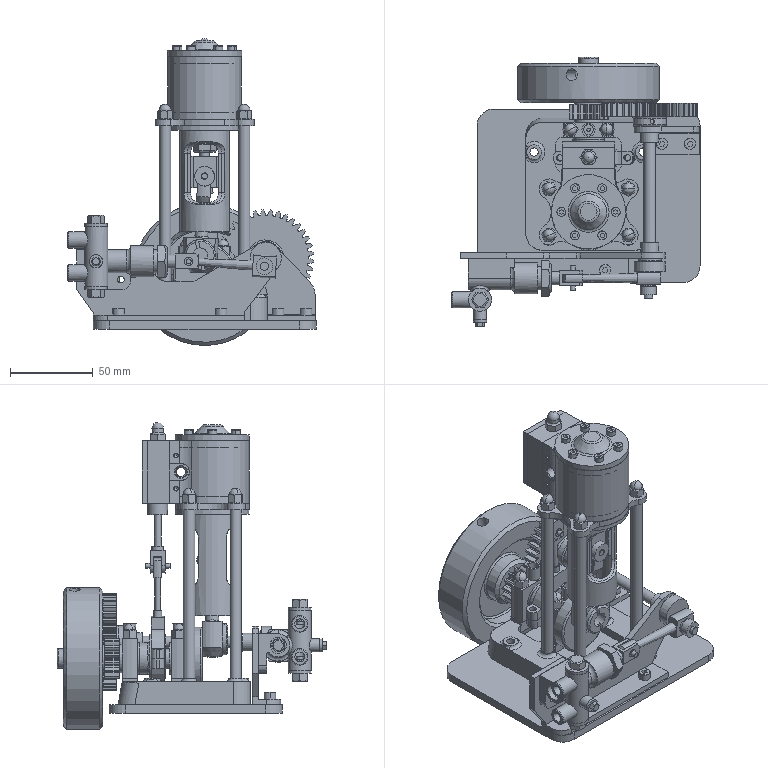Assembly | NX | mm | 88 component files | 88 solids | 1687 faces | box 150.23 x 163.5 x 186 mm | volume 461550 mm3 | plane 696 | cylinder 542 | other 255 | cone 98 | torus 67 | sphere 19 | spline 10 | commonest cylinder face diameters 4 x54 5 x50 51.75 x37 6 x30 14 x27 3 x24 2.5 x22 7 x21
Bill of materials:
unnamed part 1 | 1 |  | Short cylindrical disc/wheel with chamfered outer edges, an annular recess in one face, a raised central hub with a through-bore, and a small radial hole in the outer rim.
unnamed part 2 | 1 |  | Flanged cylindrical sleeve: a short tube with a larger-diameter flange at one end and a straight through-bore.
unnamed part 3 | 2 |  | Stepped hollow cylinder: a larger-diameter tube section with a rounded shoulder that steps down to a smaller-diameter section. It has a large bore at the large end and a smaller hole visible at the opposite end.
unnamed part 4 | 1 |  | Thin sheet-metal-like band formed into an open circular loop, with two parallel straight flanges extending from the opening. Each flange has an open-ended U-shaped slot between two small round holes.
unnamed part 5 | 1 |  | Semicircular saddle/arch body with a flat lug at each end and a rectangular block on top of the arch. Each end lug has a through-hole with rounded ends, and the top block has a vertical hole.
unnamed part 6 | 1 |  | Solid stepped round pin/shaft: a long central body with a smaller-diameter journal of similar length at each end, and small chamfers or rounds at the shoulders.
unnamed part 7 | 1 |  | Link/rod with a rectangular eye block at each end joined by a slightly tapered round shank. The two end blocks have through-holes of different sizes, and the larger block has a short raised ring/boss around its hole on the sides.
unnamed part 8 | 1 |  | Flat annular ring/washer with a uniform rectangular cross-section and a central through-hole.
unnamed part 9 | 1 |  | Long thin-walled tube with a short reduced-diameter spigot step at one end.
unnamed part 10 | 2 |  | Rectangular block with a large through-bore through its main face and three holes in the top face (two smaller outer holes and a larger center hole). Its short end faces are slightly curved.
unnamed part 11 | 4 |  | Cap-screw-shaped part: a cylindrical head with a hexagonal socket recess and a smaller plain cylindrical shank with a chamfered tip.
unnamed part 12 | 1 |  | Rod-end/link with a forked clevis at one end (two lugs, each with a small cross-hole) joined by a tapered shank to a block at the other end. The block has a large through-bore and a chamfered/rounded bottom.
unnamed part 13 | 1 |  | Solid stepped cylindrical shaft: a larger central cylinder with a smaller coaxial cylindrical journal at each end, roughly symmetric.
unnamed part 14 | 1 |  | Thin-walled cylindrical tube with a flat circular flange at one end. The flange has four evenly spaced small holes, and two opposite rounded-rectangle windows are cut through the tube wall.
unnamed part 15 | 1 |  | Flanged bushing: a cylindrical shank joined to a hexagonal collar, with a coaxial through bore. The outer face of the hex is chamfered or crowned.
unnamed part 16 | 1 |  | Long, slender stepped pin: a longer central cylindrical section of slightly larger diameter, with a shorter, narrower cylindrical section at each end. The ends appear rounded or chamfered.
unnamed part 17 | 4 |  | Plain solid cylindrical rod with flat ends.
unnamed part 18 | 1 |  | Circular flange plate with six evenly spaced through holes and a raised central conical boss with a flat, rounded-edge top. The underside has a shallow circular spigot or step.
unnamed part 19 | 1 |  | Flat plate with a lobed outline: four rounded corner ears, each with a larger hole, plus four smaller holes further inboard. There is a central through hole, a thin raised circular pad on the top face, and a cylindrical hub projecting from the underside.
unnamed part 20 | 1 |  | Hex-based tubular fitting: a hexagonal base with a taller cylindrical tubular boss and a coaxial through bore. The bottom edges of the hex are rounded or chamfered.
unnamed part 21 | 1 |  | Half-round saddle clamp: a semicircular band with a flat tab at each end, each tab having a through hole.
unnamed part 22 | 1 |  | Plain cylindrical tube or ring spacer with a concentric through bore and flat ends.
unnamed part 23 | 1 |  | Clevis-style block: a rectangular body with a U-shaped slot forming two prongs. The prongs have rounded ends and one coaxial cross hole through both. A cylindrical boss with an axial hole sits on the opposite face.
unnamed part 24 | 1 |  | Cylindrical housing with a large through bore and a flange at each end. Six small holes are arranged around the bore in the end face. A flat-sided block extends to one side, with a larger cross hole and two smaller holes, and there is a small notch near the bore edge on the top face.
unnamed part 25 | 1 |  | L-shaped bent-plate bracket: a rectangular base flange with two small round through-holes, and an upright arm that narrows and leans to one side, ending in a rounded lobe with one larger round through-hole.
unnamed part 26 | 1 |  | Straight-toothed spur gear with a cylindrical hub sticking out from one face and a central round bore. The hub has small radial holes.
unnamed part 27 | 1 |  | Thin-walled cylindrical tube with an elongated rounded-rectangle window cut through both walls near its middle.
unnamed part 28 | 1 |  | Spool- or pulley-like part: two equal flat circular flanges joined by a smaller-diameter cylindrical core, with a small central through-hole along the axis.
unnamed part 29 | 1 |  | Plain cylindrical ring or spacer with a large central bore and a moderate wall thickness. Its axial length is a little less than half its outer diameter.
unnamed part 30 | 1 |  | Long slender round shaft with a short cylindrical collar near one end. Beyond the collar is a stepped end section, and a small cross pin passes through the shaft near the other end, sticking out on both sides.
unnamed part 31 | 1 |  | Block-like part made of a thick rectangular plate with two parallel tapered prongs sticking out from one face, leaving a rectangular gap between them. An L-shaped shallow recess or pocket is cut into the opposite face.
unnamed part 32 | 1 |  | Plain thick-walled cylindrical ring or spacer with a central bore. Its axial length is about half its outer diameter.
unnamed part 33 | 1 |  | Stepped cylindrical pin: a larger-diameter main body with a domed end crossed by a narrow slot, and a shorter reduced-diameter spigot at the other end with a small chamfer.
unnamed part 34 | 1 |  | Thin flat rectangular plate with rounded corners and three parallel through-slots with rounded ends: a wider slot in the middle and two narrower slots above and below it.
unnamed part 35 | 6 |  | Socket-head cap-screw-shaped part: a cylindrical head with a hexagonal socket recess, and a plain cylindrical shank with a chamfered tip.
unnamed part 36 | 4 |  | Plain solid cylindrical rod with flat ends and no visible features along its length.
unnamed part 37 | 1 |  | Thick plate with rounded corners, two rounded-rectangle through windows, several counterbored through holes around the edge, and small plain holes.
unnamed part 38 | 1 |  | Prismatic block with an I/H-shaped plan profile, convex arced ends, vertical holes and a horizontal cross hole.
unnamed part 39 | 1 |  | Clevis-like fork: a cylindrical shank attached to a U-shaped yoke with two parallel prongs that have rounded ends and aligned cross holes.
unnamed part 40 | 1 |  | Pulley- or spool-like hub: a cylindrical drum between two thin flanges, with a smaller coaxial hub extension on one side, a central bore and one radial hole.
unnamed part 41 | 2 |  | Stepped axisymmetric body: a small top pin, a larger cylinder, a thin circular flange, and a hexagonal lower section with a chamfered bottom.
unnamed part 42 | 1 |  | Rectangular frame block with a large rounded-rectangle through window, four corner holes, a hole through the top edge, and a cylindrical boss below.
unnamed part 43 | 1 |  | Thin-walled cylindrical tube with a small rectangular notch in the rim at one end.
unnamed part 44 | 1 |  | Solid stepped cylindrical pin: a larger central cylinder with smaller coaxial cylindrical ends on both sides.
unnamed part 45 | 1 |  | Flat annular ring (washer-like) with a central through hole and flat faces.
unnamed part 46 | 1 |  | Stepped shaft: a hexagonal head, a thin circular collar or flange, a larger cylindrical section, and a long smaller-diameter pin with a rounded end.
unnamed part 47 | 8 |  | Hexagonal body with a hemispherical dome on top, resembling a cap-nut shape, with a chamfered lower hex edge.
unnamed part 48 | 1 |  | Slender eye rod: a flat rectangular tab with a round through hole and curved end, attached to a thin rod that steps up to a larger-diameter section at the far end.
unnamed part 49 | 1 |  | Long plain cylindrical pin with a thin circular disc flange near one end. A short, smaller stub sticks out from the other side of the flange and ends in a lipped head with a slot across it and a small central bore.
unnamed part 50 | 1 |  | Multi-branch tubular body. A vertical tube with a through bore has two parallel cylindrical stubs on one side and a side port. A horizontal tube runs from it, joined by a rectangular block section, and steps up to a larger hollow socket at its end. A flat rounded tab with one through hole sticks out near the base.
unnamed part 51 | 1 |  | Small spur gear made in one piece with a longer cylindrical hub, and a central through bore. The hub has one radial hole.
unnamed part 52 | 1 |  | Thin, nearly square rectangular flat plate with four through holes, one near each corner.
unnamed part 53 | 2 |  | Flanged cylindrical sleeve: a thin-walled tube with a thin outer flange at one end and one small radial hole through the barrel wall.
unnamed part 54 | 4 |  | Solid stepped cylindrical shaft: a long main body with a short, smaller-diameter journal at each end.
unnamed part 55 | 1 |  | Solid rectangular block with one cylindrical through hole running through its thickness, offset from the center along one face direction.
unnamed part 56 | 1 |  | L-shaped bracket bent from plate. The upright plate has an irregular profile with angled edges, a shallow recessed middle, and a rounded lug at one end holding a larger hole. A perpendicular flange along the bottom edge has two small holes.
unnamed part 57 | 2 |  | Flanged cylindrical sleeve with a fairly thick wall, a thin outer flange at one end, and one radial hole through the barrel.
unnamed part 58 | 1 |  | Thin flat rectangular plate with rounded corners and seven through holes of at least two sizes in an irregular, asymmetric pattern.
unnamed part 59 | 1 |  | Solid body made of a hexagonal prism with a domed (acorn-style) cylindrical cap on top and a plain cylindrical shank below.
Mates:
1. fix | Bottom_Plate 1 component
2. concentric | Base 1 edge | Bottom_Plate 1 edge
3. parallel | Base 1 face | Bottom_Plate 1 face
4. concentric | Side_Plate 1 edge | Bottom_Plate 1 edge
5. parallel | Side_Plate 1 face | Bottom_Plate 1 face
6. concentric | Bottom_Plate 1 edge | Right_Side_Plate 1 edge
7. parallel | Right_Side_Plate 1 face | Bottom_Plate 1 face
8. concentric | bearing 2 edge | Side_Plate 1 edge
9. concentric | bearing 1 edge | Right_Side_Plate 1 edge
10. concentric | column 4 edge | Base 1 edge
11. concentric | column 3 edge | Base 1 edge
12. concentric | column 2 edge | Base 1 edge
13. concentric | column 1 edge | Base 1 edge
14. concentric | Upper_Support_Plate 1 arc | column 4 edge
15. concentric | Upper_Support_Plate 1 arc | column 2 edge
16. concentric | stud 4 edge | Base 1 edge
17. concentric | stud 3 edge | Base 1 edge
18. concentric | stud 2 edge | Base 1 edge
19. concentric | stud 1 edge | Base 1 edge
20. concentric | pedestal 2 edge | Base 1 edge
21. parallel | pedestal 2 face | Base 1 face
22. concentric | pedestal 1 | Base 1 edge
23. parallel | pedestal 1 face | Base 1 face
24. touch align | pedestal_bearing 2 face | pedestal 2 face
25. touch align | pedestal_bearing 2 face | pedestal 2 face
26. touch align | pedestal_bearing 1 face | pedestal 1 face
27. touch align | pedestal_bearing 1 face | pedestal 1 face
28. concentric | vent_plug 2 edge | pedestal 2 edge
29. concentric | vent_plug 1 edge | pedestal 1 edge
30. concentric | Upper_Piston_Cylinder 1 edge | Upper_Support_Plate 1 edge
31. parallel | Upper_Piston_Cylinder 1 face | pedestal 2 face
32. concentric | Upper_Piston_Cylinder_Liner 1 edge | Upper_Piston_Cylinder 1 edge
33. parallel | Upper_Piston_Cylinder_Liner 1 face | Upper_Piston_Cylinder 1 face
34. concentric | Outer_Guard_Plate 1 edge | Upper_Piston_Cylinder 1 edge
35. parallel | Outer_Guard_Plate 1 face | Upper_Support_Plate 1 face
36. concentric | Upper_Piston_Cylinder 1 edge | end_cap 1 edge
37. concentric | end_cap 1 edge | Outer_Guard_Plate 1 edge
38. concentric | Shim_Plate 1 edge | Upper_Piston_Cylinder 1 edge
39. parallel | Shim_Plate 1 face | Upper_Piston_Cylinder 1 face
40. concentric | Upper_Piston_Cylinder 1 edge | Outer_Connecting_Block 1 edge
41. parallel | Outer_Connecting_Block 1 face | Upper_Piston_Cylinder 1 face
42. concentric | Outer_Cover_Plate 1 arc | Outer_Connecting_Block 1 edge
43. parallel | Outer_Cover_Plate 1 face | Outer_Connecting_Block 1 face
44. concentric | Outer_Connecting_Block 1 edge | Upper_Connecting_Nut 1 edge
45. parallel | Upper_Connecting_Nut 1 face | Outer_Cover_Plate 1 face
46. concentric | Small_Washer 1 arc | Outer_Connecting_Block 1 edge
47. concentric | Large_Washer 1 arc | Outer_Connecting_Block 1 edge
48. concentric | stud_M4 4 edge | Outer_Cover_Plate 1 edge
49. concentric | stud_M4 3 edge | Outer_Cover_Plate 1 edge
50. concentric | stud_M4 2 edge | Outer_Cover_Plate 1 edge
51. concentric | stud_M4 1 edge | Outer_Cover_Plate 1 edge
52. touch align | gear_shaft 1 face | flywheel 1 face
53. touch align | gear_shaft 1 face | flywheel 1 face
54. touch align | gear_shaft 1 face | Crankshaft 1 face
55. touch align | Crankshaft 1 face | pedestal_bearing 2 face
56. concentric | Piston_Ring 1 arc | Piston 1 edge
57. concentric | conn_rod 1 edge | Piston 1 arc
58. concentric | piston_conn_block 1 arc | conn_rod 1 edge
59. concentric | Lower_Piston_Cylinder 1 arc | Upper_Support_Plate 1 edge
60. concentric | Lower_Piston_Cylinder 1 edge | Upper_Support_Plate 1 edge
61. concentric | Lower_Piston_Cylinder_Liner 1 edge | Lower_Piston_Cylinder 1 edge
62. parallel | Lower_Piston_Cylinder_Liner 1 face | Lower_Piston_Cylinder 1 face
63. touch align | conn_rod 1 face | Upper_Support_Plate 1 face
64. parallel | piston_conn_block 1 face | Side_Plate 1 face
65. concentric | Bottom_Plate_Connecting_Ring 1 edge | Upper_Support_Plate 1 edge
66. concentric | Bottom_Plate_Washer 1 arc | Bottom_Plate_Connecting_Ring 1 edge
67. concentric | Bottom_Plate_Connecting_Screw 1 edge | Bottom_Plate_Washer 1 edge
68. parallel | Bottom_Plate_Connecting_Screw 1 face | Side_Plate 1 face
69. concentric | conn_pin 1 edge | Piston_Rod_Connecting_Shaft 1 edge
70. touch align | Piston_Rod_Connecting_Shaft 1 face | Crankshaft 1 face
71. touch align | conn_pin 1 face | piston_conn_block 1 face
72. center | Piston_Rod_Connecting_Shaft 1 face | Piston_Rod_Connecting_Shaft 1 face | piston_conn_block 1 face | piston_conn_block 1 face
73. touch align | Large_Gear_Shaft 1 face | Large_Gear 1 face
74. touch align | Large_Gear_Shaft 1 face | Large_Gear 1 face
75. touch align | Large_Gear_Shaft 1 face | bearing 1 face
76. center | Crankshaft 1 face | Crankshaft 1 face | Piston_Rod_Connecting_Shaft 1 face | Piston_Rod_Connecting_Shaft 1 face
77. center | Eccentric_Shaft 1 face | Eccentric_Shaft 1 face | Outer_Connecting_Block 1 face
78. concentric | Lower_Piston_Connecting_Rod 1 arc | Upper_Piston_Ring 1 edge
79. parallel | Upper_Piston_Ring 1 face | Lower_Piston_Connecting_Rod 1 face
80. concentric | piston_conn_rod 1 edge | Upper_Piston_Ring 1 edge
81. parallel | piston_conn_rod 1 face | Upper_Piston_Ring 1 face
82. touch align | Lower_Piston_Connecting_Rod 1 face | Eccentric_Shaft 1 face
83. center | Lower_Piston_Connecting_Rod 1 face | Lower_Piston_Connecting_Rod 1 face | Eccentric_Shaft 1 face | Eccentric_Shaft 1 face
84. concentric | conn_shaft_1 1 edge | conn_block 1 arc
85. concentric | conn_shaft 1 edge | conn_block 1 edge
86. touch align | slider_baffle 1 face | slider 1 face
87. touch align | slider_baffle 1 face | slider 1 face
88. center | slider_baffle 1 face | slider_baffle 1 face | slider 1 face | slider 1 face
89. touch align | slider_baffle 1 face | conn_shaft_1 1 face
90. parallel | slider 1 face | conn_block 1 face
91. distance | slider 1 face | conn_shaft 1 face
92. touch align | piston_conn_rod 1 face | conn_shaft 1 face
93. center | conn_block 1 face | conn_block 1 face | piston_conn_rod 1 face | piston_conn_rod 1 face
94. touch align | conn_shaft_1 1 face | Outer_Connecting_Block 1 face
95. bond | Eccentric_Shaft 1 component | Crankshaft 1 component
96. concentric | Outer_Casing_Tube 1 edge | Side_Plate 1 edge
97. parallel | Outer_Casing_Tube 1 face | Side_Plate 1 face
98. concentric | Piston_Straight_Rod_Connecting_Block 1 edge | Piston_Straight_Rod 1 arc
99. concentric | Piston_Straight_Rod_Connecting_Pin 1 edge | Piston_Straight_Rod_Connecting_Block 1 edge
100. touch align | Piston_Straight_Rod 1 face | Outer_Casing_Tube 1 face
101. parallel | Piston_Straight_Rod_Connecting_Block 1 face | Side_Plate 1 face
102. touch align | Outer_Casing_Tube_Connecting_Rod 1 face | Piston_Straight_Rod_Connecting_Pin 1 face
103. center | Outer_Casing_Tube_Connecting_Rod 1 face | Outer_Casing_Tube_Connecting_Rod 1 face | Piston_Straight_Rod_Connecting_Block 1 face | Piston_Straight_Rod_Connecting_Block 1 face
104. touch align | Outer_Casing_Tube_Connecting_Rod 1 face | Large_Gear_Shaft 1 face
105. touch align | Large_Gear 1 face | Right_Side_Plate 1 face
106. concentric | Outer_Casing_Tube_Washer 1 arc | Outer_Casing_Tube 1 edge
107. concentric | Outer_Casing_Tube_Connecting_Screw 1 edge | Outer_Casing_Tube_Washer 1 edge
108. parallel | Outer_Casing_Tube_Connecting_Screw 1 face | Side_Plate 1 face
109. concentric | arm_tube_nut 2 edge | Outer_Casing_Tube 1 edge
110. concentric | arm_tube_nut 1 edge | Outer_Casing_Tube 1 edge
111. concentric | Outer_Casing_Tube_Small_Bolt 1 edge | Outer_Casing_Tube 1 edge
112. parallel | Outer_Casing_Tube_Small_Bolt 1 face | Side_Plate 1 face
113. concentric | Upper_Support_Plate 1 edge | GB_T_802_1_Combined_Cap_Nut_M5 8
114. concentric | GB_T_802_1_Combined_Cap_Nut_M5 7 | Upper_Support_Plate 1 edge
115. concentric | GB_T_802_1_Combined_Cap_Nut_M5 6 | Upper_Support_Plate 1 edge
116. concentric | GB_T_802_1_Combined_Cap_Nut_M5 5 | Upper_Support_Plate 1 edge
117. concentric | GB_T_802_1_Combined_Cap_Nut_M5 4 | pedestal 1
118. parallel | GB_T_802_1_Combined_Cap_Nut_M5 4 face | Base 1 face
119. concentric | GB_T_802_1_Combined_Cap_Nut_M5 3 | pedestal 1
120. parallel | GB_T_802_1_Combined_Cap_Nut_M5 3 face | Base 1 face
121. concentric | GB_T_802_1_Combined_Cap_Nut_M5 2 edge | pedestal 2 edge
122. parallel | GB_T_802_1_Combined_Cap_Nut_M5 2 face | Right_Side_Plate 1 face
123. concentric | GB_T_802_1_Combined_Cap_Nut_M5 1 | pedestal 2 edge
124. parallel | GB_T_802_1_Combined_Cap_Nut_M5 1 face | pedestal 2 face
125. concentric | GB_T_70_1_Hex_Socket_Cap_Screw_M3x10 6 edge | end_cap 1 edge
126. bond | end_cap 1 component | assembly component
127. bond | GB_T_70_1_Hex_Socket_Cap_Screw_M3x10 6 component | assembly component
128. bond | GB_T_70_1_Hex_Socket_Cap_Screw_M3x10 5 component | assembly component
129. bond | GB_T_70_1_Hex_Socket_Cap_Screw_M3x10 4 component | assembly component
130. bond | GB_T_70_1_Hex_Socket_Cap_Screw_M3x10 3 component | assembly component
131. circular | assembly datumaxis | assembly cartesiancoordinatesystem | assembly cartesiancoordinatesystem | assembly cartesiancoordinatesystem | assembly cartesiancoordinatesystem | assembly cartesiancoordinatesystem | assembly cartesiancoordinatesystem
132. bond | GB_T_70_1_Hex_Socket_Cap_Screw_M3x10 2 component | assembly component
133. bond | GB_T_70_1_Hex_Socket_Cap_Screw_M3x10 1 component | assembly component
134. concentric | GB_T_70_1_Hex_Socket_Cap_Screw_M4x8 4 edge | Side_Plate 1 edge
135. concentric | GB_T_70_1_Hex_Socket_Cap_Screw_M4x8 3 edge | Side_Plate 1 edge
136. concentric | GB_T_70_1_Hex_Socket_Cap_Screw_M4x8 2 edge | Right_Side_Plate 1 edge
137. concentric | GB_T_70_1_Hex_Socket_Cap_Screw_M4x8 1 edge | Right_Side_Plate 1 edge